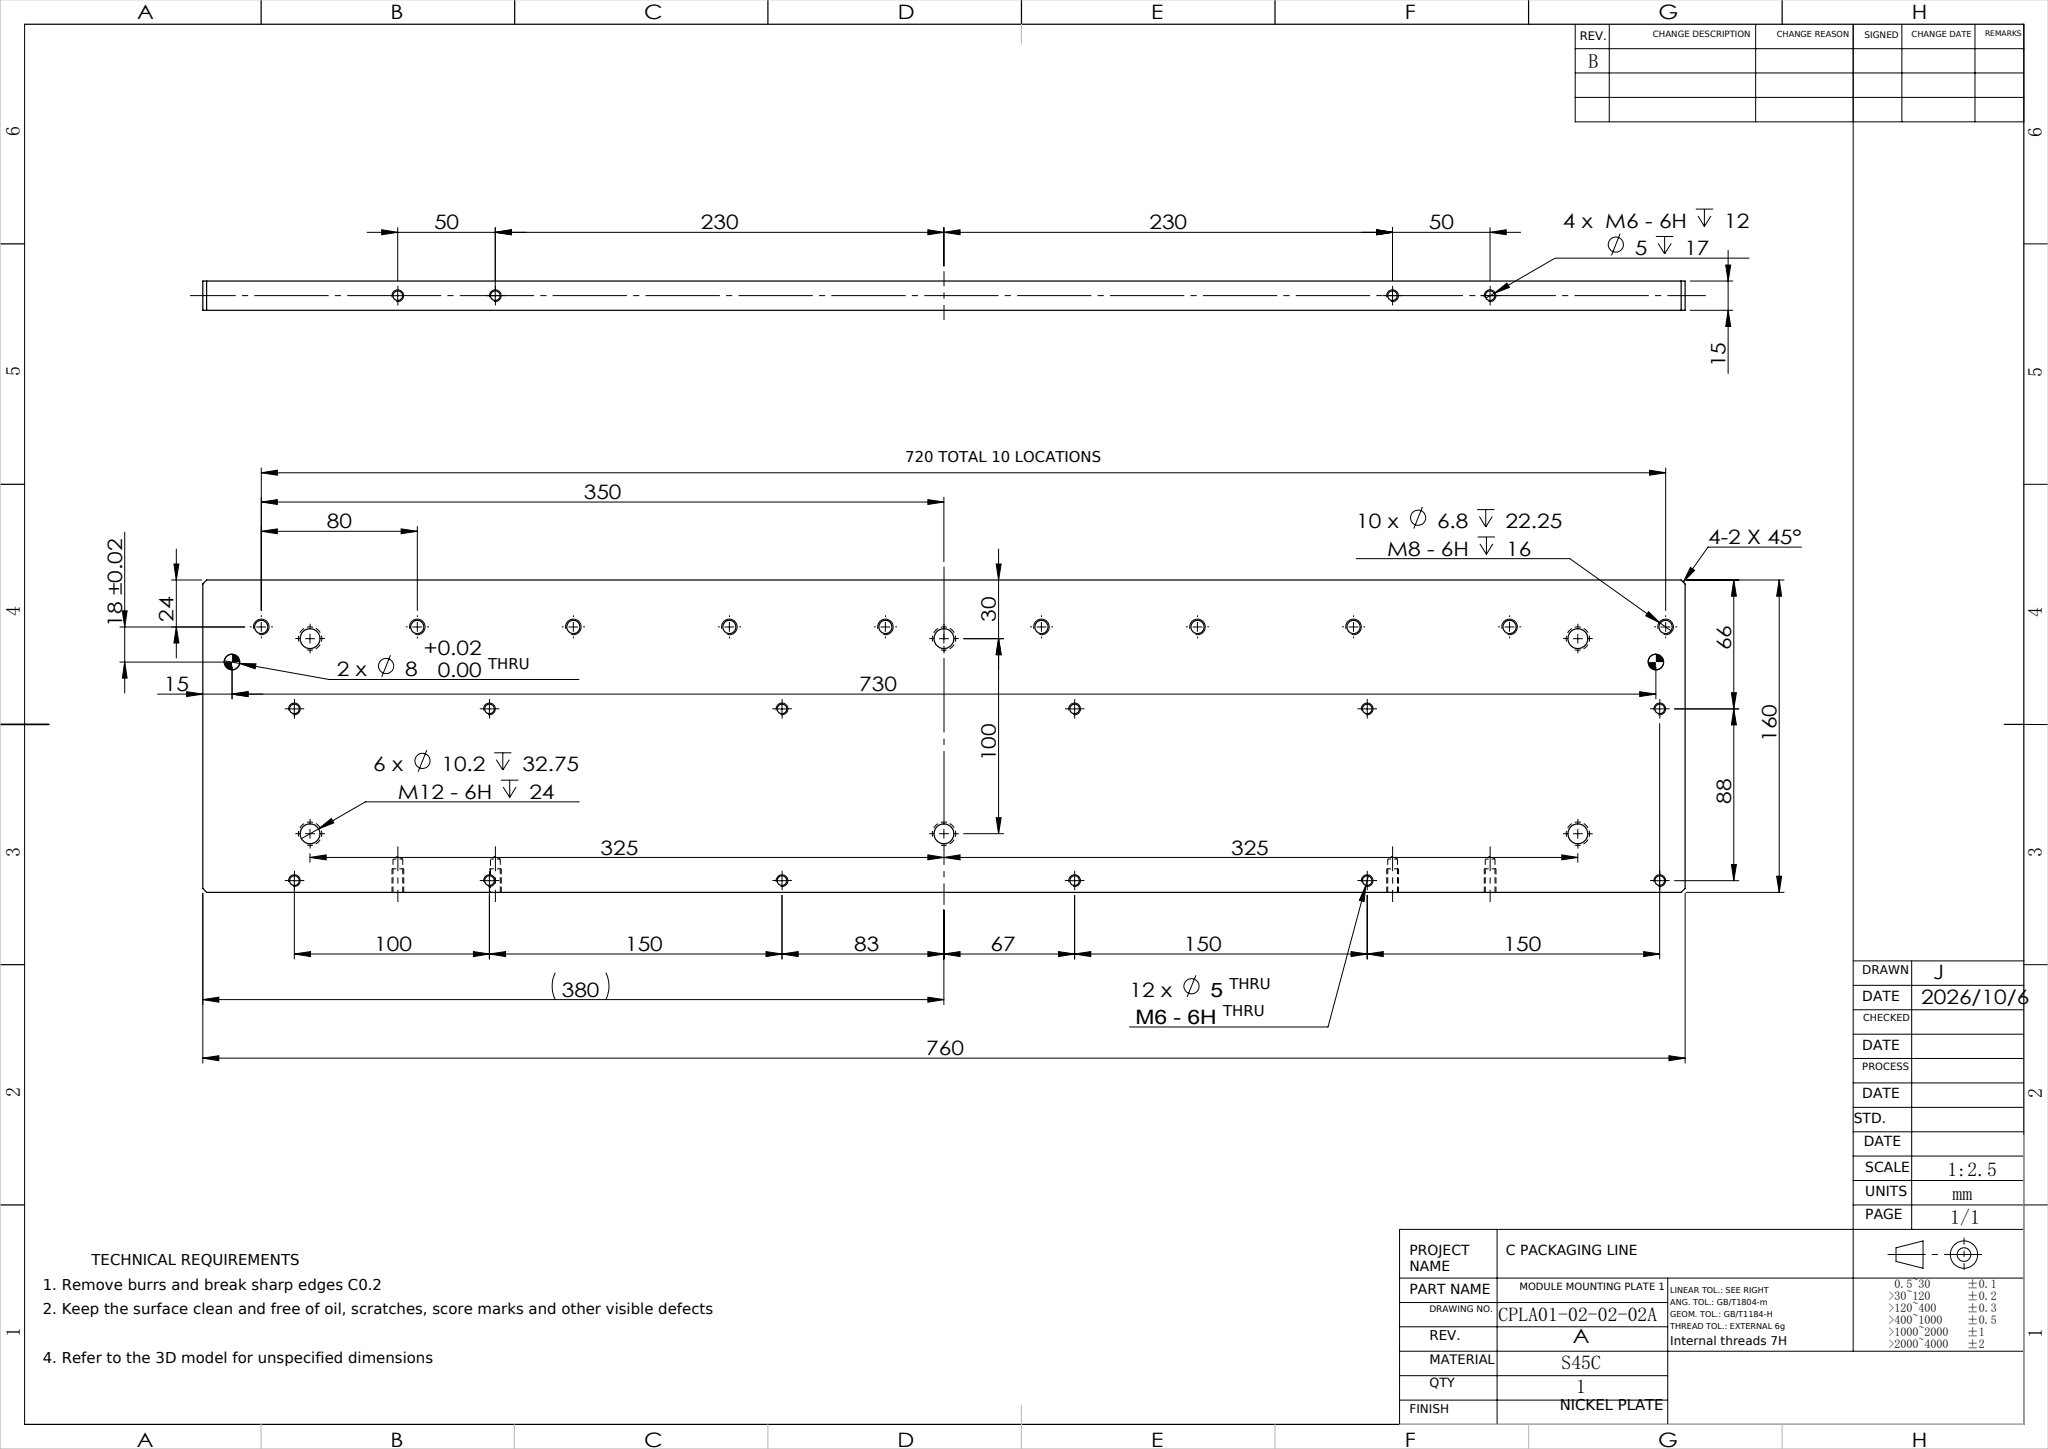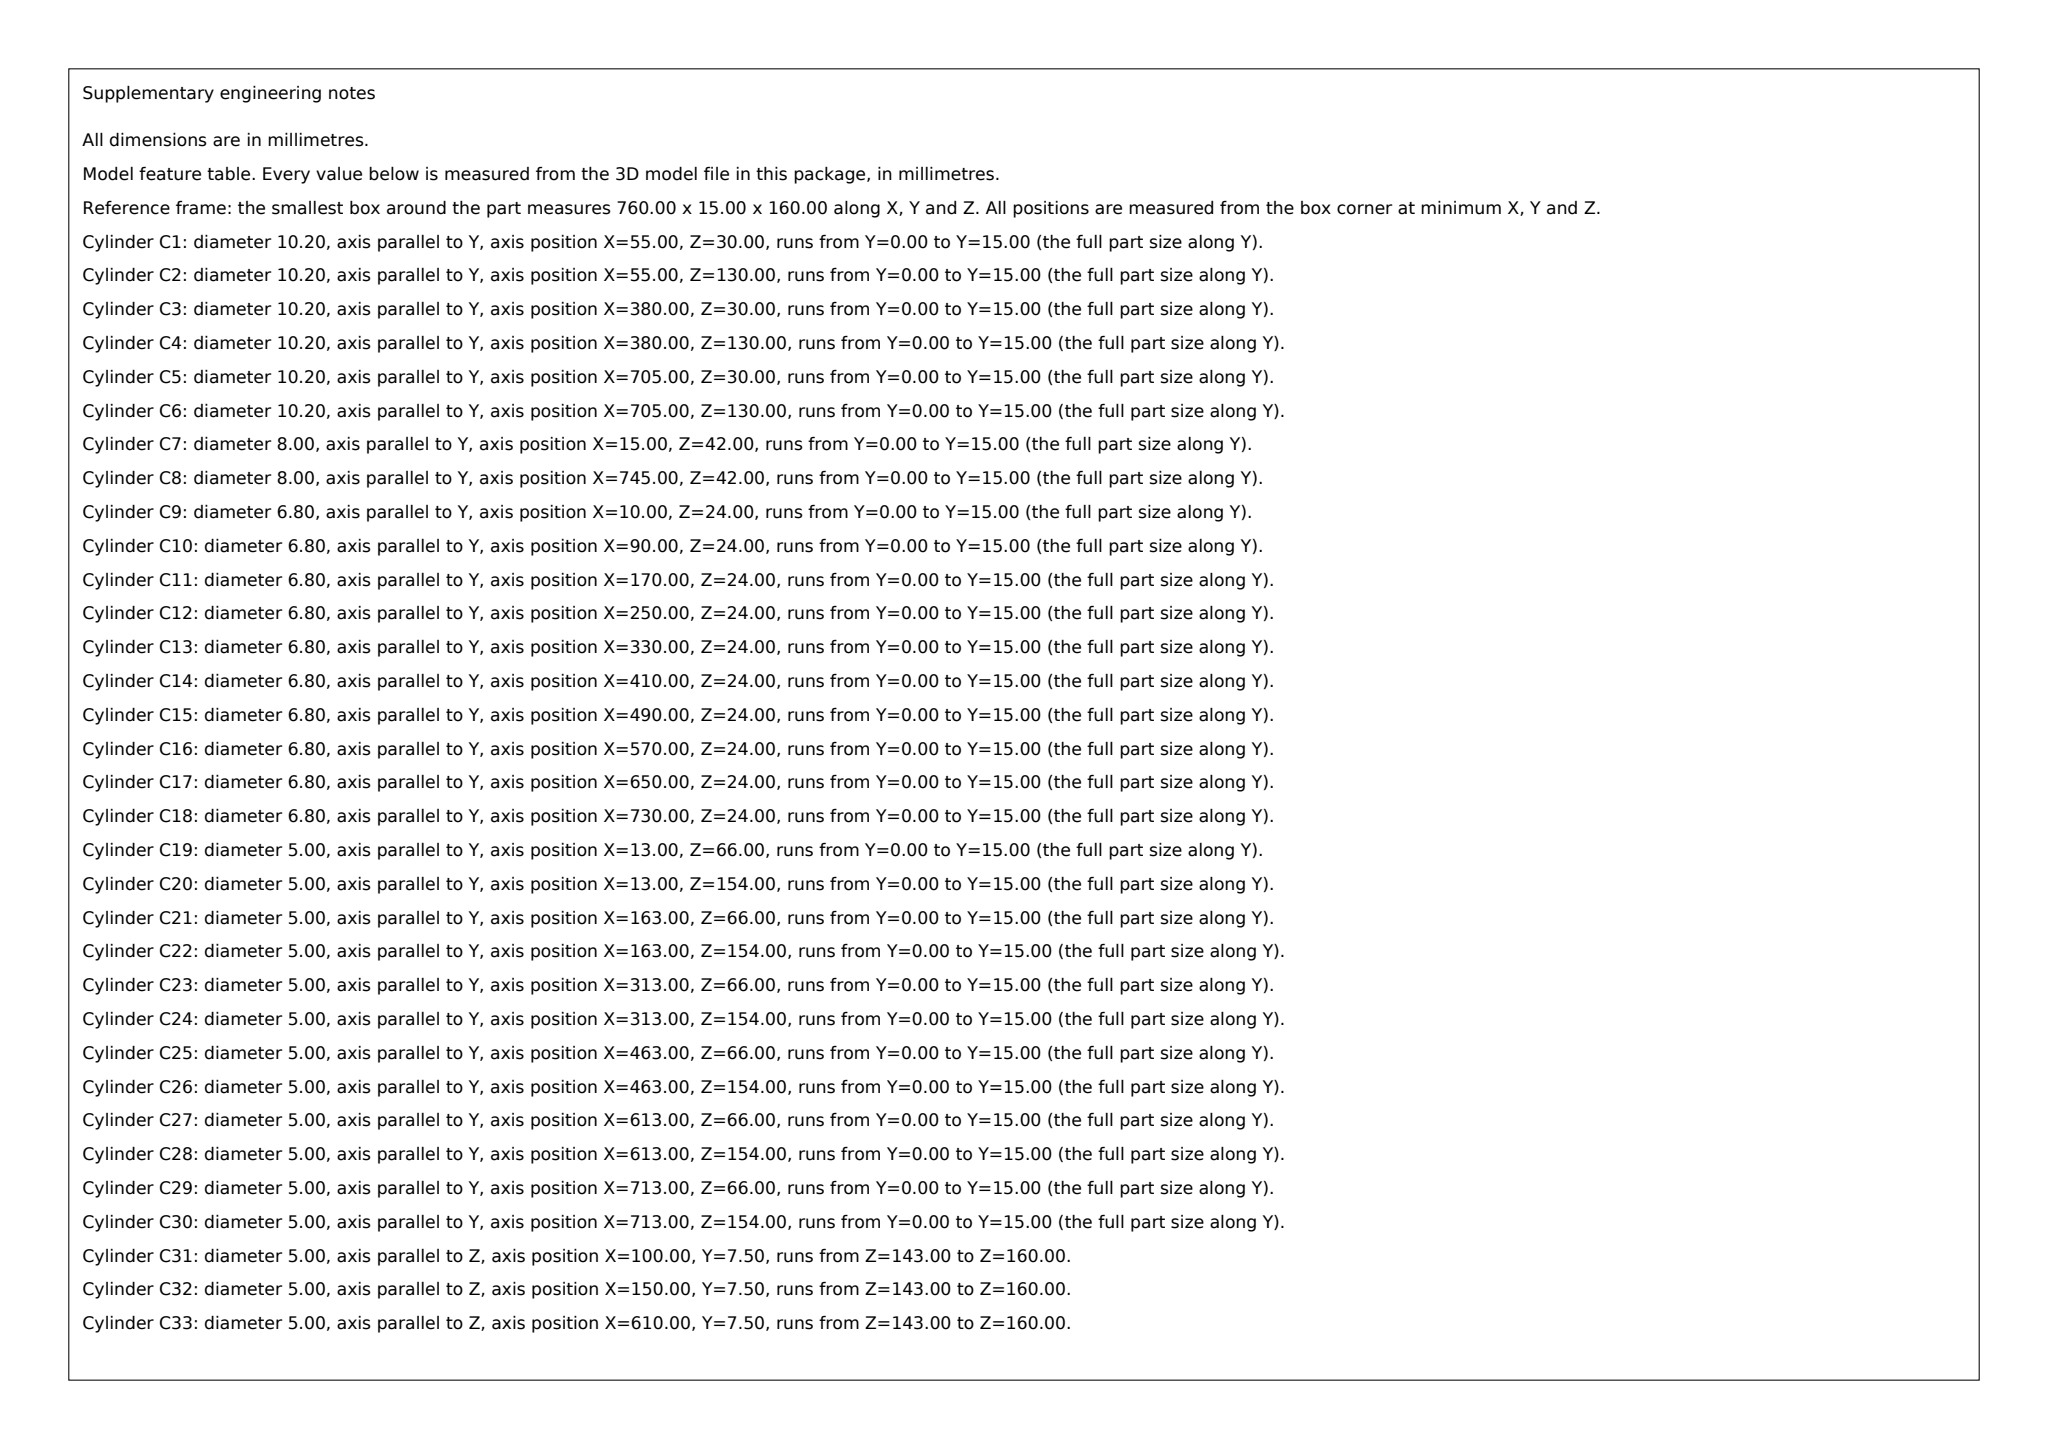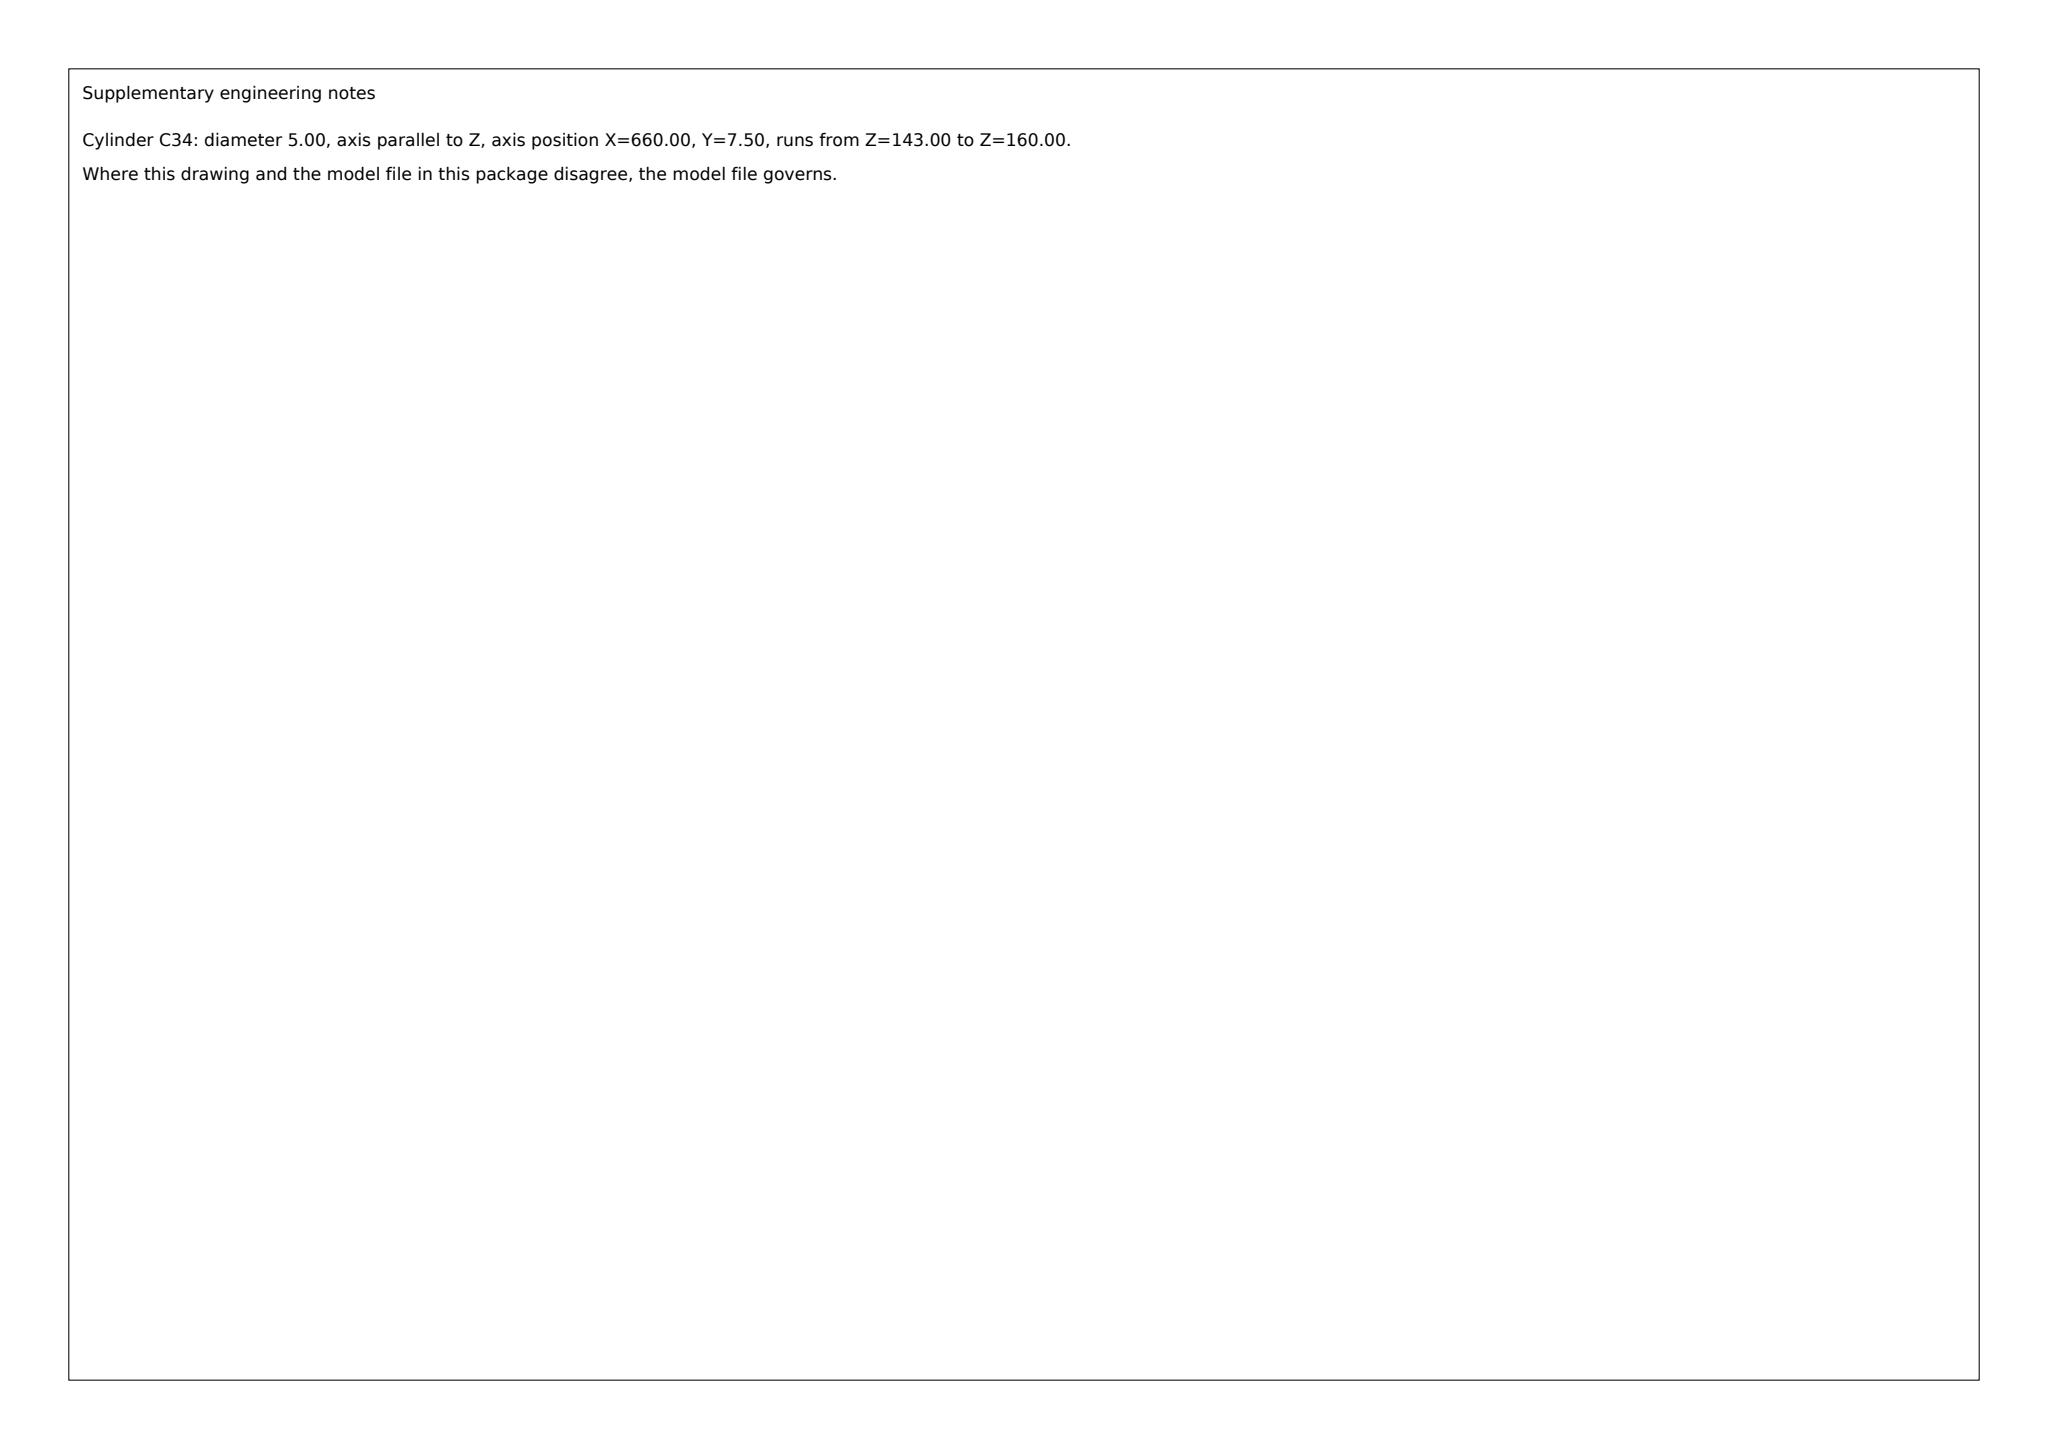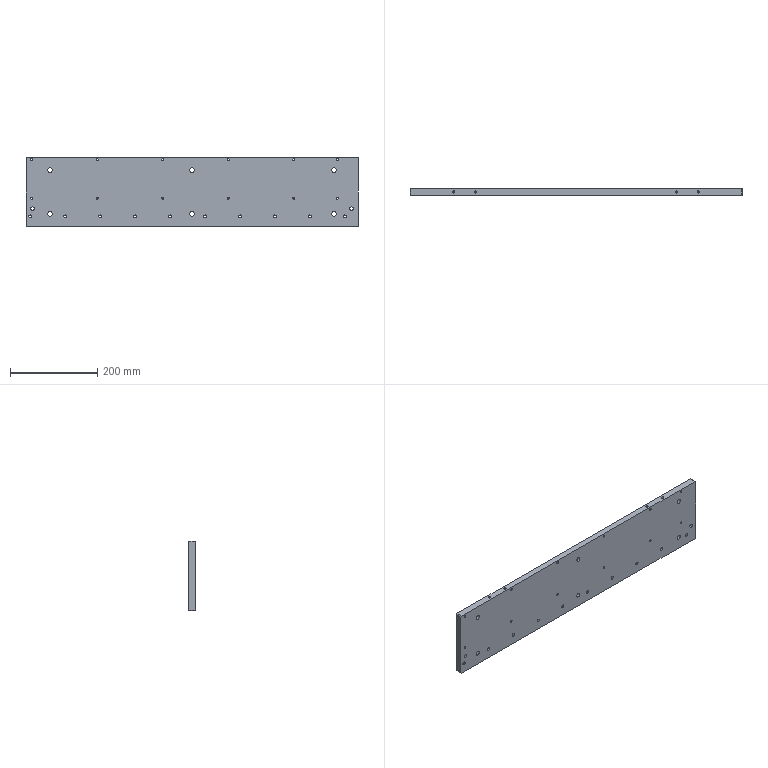Part | SolidWorks | mm | material S45C | 1 solid | 86 faces | box 760 x 15 x 160 mm | volume 1804687 mm3 | cylinder 68 | plane 10 | cone 8 | commonest cylinder face diameters 5 x32 6.8 x20 10.2 x12 8 x4
build123d program:
from build123d import *

# Parameters (mm, degrees)
SKETCH1_W                 = 760
SKETCH1_H                 = 160
BOSS_EXTRUDE1_DEPTH       = 15
M12_TAPPED_HOLE1_D        = 10.2
M12_TAPPED_HOLE1_DEPTH    = 32.75
M12_TAPPED_HOLE1_TIP      = 3.064
M8_TAPPED_HOLE1_D         = 6.8
M8_TAPPED_HOLE1_DEPTH     = 22.25
M8_TAPPED_HOLE1_TIP       = 2.043
F_8_0MM_DOWEL_PIN_HOLE1_D = 8
M6_TAPPED_HOLE1_D         = 5
CHAMFER1_SIZE             = 2
M6_TAPPED_HOLE3_D         = 5
M6_TAPPED_HOLE3_DEPTH     = 17
M6_TAPPED_HOLE3_TIP       = 1.502


with BuildPart() as part:
    # Sketch1 → Boss-Extrude1 (new body)
    with BuildSketch(Plane(origin=(0, 0, 0), x_dir=(1, 0, 0), z_dir=(0, 1, 0))):
        Rectangle(SKETCH1_W, SKETCH1_H)
    extrude(amount=BOSS_EXTRUDE1_DEPTH)

    # M12 Tapped Hole1
    with Locations(Plane(origin=(0, 15, 0), x_dir=(1, 0, 0), z_dir=(0, 1, 0))):
        with Locations((-325, 50), (-325, -50), (0, -50), (0, 50), (325, 50), (325, -50)):
            Hole(M12_TAPPED_HOLE1_D / 2, depth=M12_TAPPED_HOLE1_DEPTH)
            with Locations((0, 0, -(M12_TAPPED_HOLE1_DEPTH + M12_TAPPED_HOLE1_TIP / 2))):  # 118° drill point
                Cone(0, M12_TAPPED_HOLE1_D / 2, M12_TAPPED_HOLE1_TIP, mode=Mode.SUBTRACT)

    # M8 Tapped Hole1
    with Locations(Plane(origin=(0, 0, 0), x_dir=(-1, 0, 0), z_dir=(0, -1, 0))):
        with Locations((-350, 56), (-270, 56), (-190, 56), (-110, 56), (-30, 56), (50, 56), (130, 56), (210, 56), (290, 56), (370, 56)):
            Hole(M8_TAPPED_HOLE1_D / 2, depth=M8_TAPPED_HOLE1_DEPTH)
            with Locations((0, 0, -(M8_TAPPED_HOLE1_DEPTH + M8_TAPPED_HOLE1_TIP / 2))):  # 118° drill point
                Cone(0, M8_TAPPED_HOLE1_D / 2, M8_TAPPED_HOLE1_TIP, mode=Mode.SUBTRACT)

    # 8.0mm Dowel Pin Hole1 (through all)
    with Locations(Plane(origin=(0, 0, 0), x_dir=(-1, 0, 0), z_dir=(0, -1, 0))):
        with Locations((-365, 38), (365, 38)):
            Hole(F_8_0MM_DOWEL_PIN_HOLE1_D / 2)

    # M6 Tapped Hole1 (through all)
    with Locations(Plane(origin=(0, 0, 0), x_dir=(-1, 0, 0), z_dir=(0, -1, 0))):
        with Locations((-333, 14), (-333, -74), (-233, -74), (-233, 14), (-83, 14), (-83, -74), (67, -74), (67, 14), (217, 14), (217, -74), (367, -74), (367, 14)):
            Hole(M6_TAPPED_HOLE1_D / 2)

    # Chamfer1
    chamfer1_edges = [part.edges().sort_by_distance(p)[0] for p in [
        (-380, 7.5, -80),
        (380, 7.5, -80),
        (380, 7.5, 80),
        (-380, 7.5, 80),
    ]]
    chamfer(chamfer1_edges, length=CHAMFER1_SIZE)

    # M6 Tapped Hole3
    with Locations(Plane.XY.offset(80)):
        with Locations((280, 7.5), (230, 7.5), (-230, 7.5), (-280, 7.5)):
            Hole(M6_TAPPED_HOLE3_D / 2, depth=M6_TAPPED_HOLE3_DEPTH)
            with Locations((0, 0, -(M6_TAPPED_HOLE3_DEPTH + M6_TAPPED_HOLE3_TIP / 2))):  # 118° drill point
                Cone(0, M6_TAPPED_HOLE3_D / 2, M6_TAPPED_HOLE3_TIP, mode=Mode.SUBTRACT)


solid = part.part